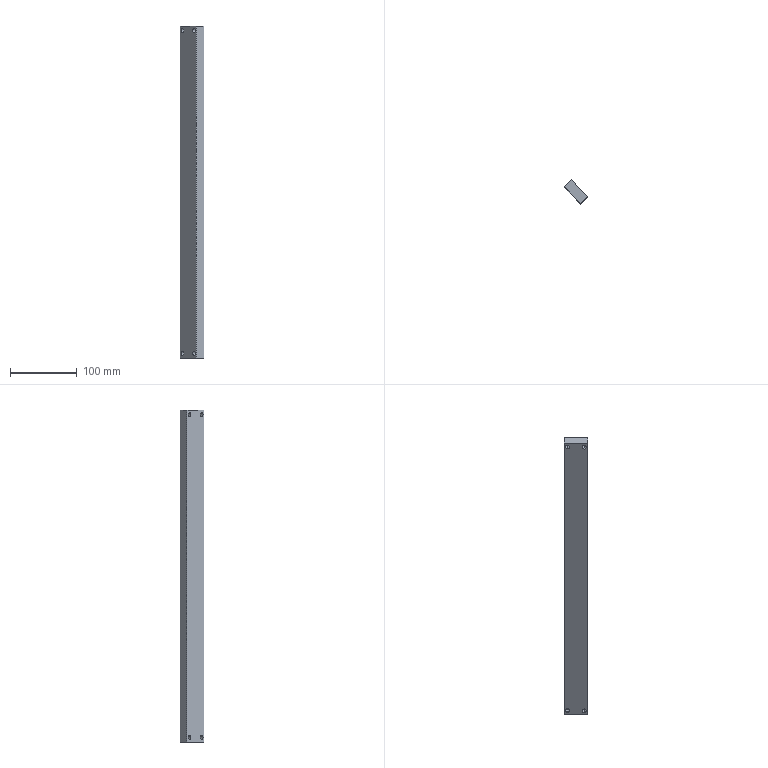Component | SolidWorks | ConnectingPlate-1 | 1 solid | 14 faces | box 34.91 x 35.77 x 499 mm | volume 259984 mm3 | cylinder 8 | plane 6 | commonest cylinder face diameters 6.5 x8
build123d program:
from build123d import *

# Parameters (mm, degrees)
SKETCH1_W           = 499
SKETCH1_H           = 35
SKETCH1_R           = 3.25
BOSS_EXTRUDE1_DEPTH = 15


with BuildPart() as part:
    # Sketch1 → Boss-Extrude1 (new body)
    with BuildSketch(Plane(origin=(0, 0, -7.5), x_dir=(-1, 0, 0), z_dir=(0, 0, -1))):
        Rectangle(SKETCH1_W, SKETCH1_H)
        with Locations(Location((-242.5, 12.5, 0), (0, 0, 180))):
            Circle(SKETCH1_R, mode=Mode.SUBTRACT)
        with Locations(Location((242.5, 12.5, 0), (0, 0, 180))):
            Circle(SKETCH1_R, mode=Mode.SUBTRACT)
        with Locations(Location((242.5, -12.5, 0), (0, 0, 180))):
            Circle(SKETCH1_R, mode=Mode.SUBTRACT)
        with Locations(Location((-242.5, -12.5, 0), (0, 0, 180))):
            Circle(SKETCH1_R, mode=Mode.SUBTRACT)
    extrude(amount=-BOSS_EXTRUDE1_DEPTH)


solid = part.part

# Placed as in the assembly
solid = solid.moved(Location((325.391, 503.025, 0.3), (90, -46.734, 90)))
STEP:
#1=COLOUR_RGB('',0.7922,0.8196,0.9333);
#2=FILL_AREA_STYLE_COLOUR('',#1);
#3=FILL_AREA_STYLE('',(#2));
#4=SURFACE_STYLE_FILL_AREA(#3);
#5=SURFACE_SIDE_STYLE('',(#4));
#6=SURFACE_STYLE_USAGE(.BOTH.,#5);
#7=PRESENTATION_STYLE_ASSIGNMENT((#6));
#8=CARTESIAN_POINT('',(12.933,19.243,9.687));
#9=VERTEX_POINT('',#8);
#10=CARTESIAN_POINT('',(12.933,19.243,9.431));
#11=VERTEX_POINT('',#10);
#12=CARTESIAN_POINT('',(12.933,19.243,9.559));
#13=DIRECTION('',(0.7282,0.6854,-0.));
#14=DIRECTION('',(0.,0.,1.));
#15=AXIS2_PLACEMENT_3D('',#12,#13,#14);
#16=CIRCLE('',#15,0.128);
#17=EDGE_CURVE('',#9,#11,#16,.T.);
#18=ORIENTED_EDGE('',*,*,#17,.F.);
#19=CARTESIAN_POINT('',(13.363,19.648,9.687));
#20=VERTEX_POINT('',#19);
#21=CARTESIAN_POINT('',(12.933,19.243,9.687));
#22=DIRECTION('',(0.7282,0.6854,-0.));
#23=VECTOR('',#22,39.37);
#24=LINE('',#21,#23);
#25=EDGE_CURVE('',#9,#20,#24,.T.);
#26=ORIENTED_EDGE('',*,*,#25,.T.);
#27=CARTESIAN_POINT('',(13.363,19.648,9.431));
#28=VERTEX_POINT('',#27);
#29=CARTESIAN_POINT('',(13.363,19.648,9.559));
#30=DIRECTION('',(0.7282,0.6854,-0.));
#31=DIRECTION('',(0.,0.,1.));
#32=AXIS2_PLACEMENT_3D('',#29,#30,#31);
#33=CIRCLE('',#32,0.128);
#34=EDGE_CURVE('',#20,#28,#33,.T.);
#35=ORIENTED_EDGE('',*,*,#34,.T.);
#36=CARTESIAN_POINT('',(12.933,19.243,9.431));
#37=DIRECTION('',(0.7282,0.6854,-0.));
#38=VECTOR('',#37,39.37);
#39=LINE('',#36,#38);
#40=EDGE_CURVE('',#11,#28,#39,.T.);
#41=ORIENTED_EDGE('',*,*,#40,.F.);
#42=EDGE_LOOP('',(#18,#26,#35,#41));
#43=FACE_OUTER_BOUND('',#42,.T.);
#44=CARTESIAN_POINT('',(12.933,19.243,9.559));
#45=DIRECTION('',(0.7282,0.6854,-0.));
#46=DIRECTION('',(0.,0.,-1.));
#47=AXIS2_PLACEMENT_3D('',#44,#45,#46);
#48=CYLINDRICAL_SURFACE('',#47,0.128);
#49=ADVANCED_FACE('',(#43),#48,.F.);
#50=CARTESIAN_POINT('',(12.933,19.243,-9.407));
#51=VERTEX_POINT('',#50);
#52=CARTESIAN_POINT('',(12.933,19.243,-9.663));
#53=VERTEX_POINT('',#52);
#54=CARTESIAN_POINT('',(12.933,19.243,-9.535));
#55=DIRECTION('',(0.7282,0.6854,-0.));
#56=DIRECTION('',(0.,0.,1.));
#57=AXIS2_PLACEMENT_3D('',#54,#55,#56);
#58=CIRCLE('',#57,0.128);
#59=EDGE_CURVE('',#51,#53,#58,.T.);
#60=ORIENTED_EDGE('',*,*,#59,.F.);
#61=CARTESIAN_POINT('',(13.363,19.648,-9.407));
#62=VERTEX_POINT('',#61);
#63=CARTESIAN_POINT('',(12.933,19.243,-9.407));
#64=DIRECTION('',(0.7282,0.6854,-0.));
#65=VECTOR('',#64,39.37);
#66=LINE('',#63,#65);
#67=EDGE_CURVE('',#51,#62,#66,.T.);
#68=ORIENTED_EDGE('',*,*,#67,.T.);
#69=CARTESIAN_POINT('',(13.363,19.648,-9.663));
#70=VERTEX_POINT('',#69);
#71=CARTESIAN_POINT('',(13.363,19.648,-9.535));
#72=DIRECTION('',(0.7282,0.6854,-0.));
#73=DIRECTION('',(0.,0.,1.));
#74=AXIS2_PLACEMENT_3D('',#71,#72,#73);
#75=CIRCLE('',#74,0.128);
#76=EDGE_CURVE('',#62,#70,#75,.T.);
#77=ORIENTED_EDGE('',*,*,#76,.T.);
#78=CARTESIAN_POINT('',(12.933,19.243,-9.663));
#79=DIRECTION('',(0.7282,0.6854,-0.));
#80=VECTOR('',#79,39.37);
#81=LINE('',#78,#80);
#82=EDGE_CURVE('',#53,#70,#81,.T.);
#83=ORIENTED_EDGE('',*,*,#82,.F.);
#84=EDGE_LOOP('',(#60,#68,#77,#83));
#85=FACE_OUTER_BOUND('',#84,.T.);
#86=CARTESIAN_POINT('',(12.933,19.243,-9.535));
#87=DIRECTION('',(0.7282,0.6854,-0.));
#88=DIRECTION('',(0.,0.,-1.));
#89=AXIS2_PLACEMENT_3D('',#86,#87,#88);
#90=CYLINDRICAL_SURFACE('',#89,0.128);
#91=ADVANCED_FACE('',(#85),#90,.F.);
#92=CARTESIAN_POINT('',(12.258,19.96,-9.407));
#93=VERTEX_POINT('',#92);
#94=CARTESIAN_POINT('',(12.258,19.96,-9.663));
#95=VERTEX_POINT('',#94);
#96=CARTESIAN_POINT('',(12.258,19.96,-9.535));
#97=DIRECTION('',(0.7282,0.6854,-0.));
#98=DIRECTION('',(0.,0.,1.));
#99=AXIS2_PLACEMENT_3D('',#96,#97,#98);
#100=CIRCLE('',#99,0.128);
#101=EDGE_CURVE('',#93,#95,#100,.T.);
#102=ORIENTED_EDGE('',*,*,#101,.F.);
#103=CARTESIAN_POINT('',(12.688,20.365,-9.407));
#104=VERTEX_POINT('',#103);
#105=CARTESIAN_POINT('',(12.258,19.96,-9.407));
#106=DIRECTION('',(0.7282,0.6854,-0.));
#107=VECTOR('',#106,39.37);
#108=LINE('',#105,#107);
#109=EDGE_CURVE('',#93,#104,#108,.T.);
#110=ORIENTED_EDGE('',*,*,#109,.T.);
#111=CARTESIAN_POINT('',(12.688,20.365,-9.663));
#112=VERTEX_POINT('',#111);
#113=CARTESIAN_POINT('',(12.688,20.365,-9.535));
#114=DIRECTION('',(0.7282,0.6854,-0.));
#115=DIRECTION('',(0.,0.,1.));
#116=AXIS2_PLACEMENT_3D('',#113,#114,#115);
#117=CIRCLE('',#116,0.128);
#118=EDGE_CURVE('',#104,#112,#117,.T.);
#119=ORIENTED_EDGE('',*,*,#118,.T.);
#120=CARTESIAN_POINT('',(12.258,19.96,-9.663));
#121=DIRECTION('',(0.7282,0.6854,-0.));
#122=VECTOR('',#121,39.37);
#123=LINE('',#120,#122);
#124=EDGE_CURVE('',#95,#112,#123,.T.);
#125=ORIENTED_EDGE('',*,*,#124,.F.);
#126=EDGE_LOOP('',(#102,#110,#119,#125));
#127=FACE_OUTER_BOUND('',#126,.T.);
#128=CARTESIAN_POINT('',(12.258,19.96,-9.535));
#129=DIRECTION('',(0.7282,0.6854,-0.));
#130=DIRECTION('',(0.,0.,-1.));
#131=AXIS2_PLACEMENT_3D('',#128,#129,#130);
#132=CYLINDRICAL_SURFACE('',#131,0.128);
#133=ADVANCED_FACE('',(#127),#132,.F.);
#134=CARTESIAN_POINT('',(12.258,19.96,9.687));
#135=VERTEX_POINT('',#134);
#136=CARTESIAN_POINT('',(12.258,19.96,9.431));
#137=VERTEX_POINT('',#136);
#138=CARTESIAN_POINT('',(12.258,19.96,9.559));
#139=DIRECTION('',(0.7282,0.6854,-0.));
#140=DIRECTION('',(0.,0.,1.));
#141=AXIS2_PLACEMENT_3D('',#138,#139,#140);
#142=CIRCLE('',#141,0.128);
#143=EDGE_CURVE('',#135,#137,#142,.T.);
#144=ORIENTED_EDGE('',*,*,#143,.F.);
#145=CARTESIAN_POINT('',(12.688,20.365,9.687));
#146=VERTEX_POINT('',#145);
#147=CARTESIAN_POINT('',(12.258,19.96,9.687));
#148=DIRECTION('',(0.7282,0.6854,-0.));
#149=VECTOR('',#148,39.37);
#150=LINE('',#147,#149);
#151=EDGE_CURVE('',#135,#146,#150,.T.);
#152=ORIENTED_EDGE('',*,*,#151,.T.);
#153=CARTESIAN_POINT('',(12.688,20.365,9.431));
#154=VERTEX_POINT('',#153);
#155=CARTESIAN_POINT('',(12.688,20.365,9.559));
#156=DIRECTION('',(0.7282,0.6854,-0.));
#157=DIRECTION('',(0.,0.,1.));
#158=AXIS2_PLACEMENT_3D('',#155,#156,#157);
#159=CIRCLE('',#158,0.128);
#160=EDGE_CURVE('',#146,#154,#159,.T.);
#161=ORIENTED_EDGE('',*,*,#160,.T.);
#162=CARTESIAN_POINT('',(12.258,19.96,9.431));
#163=DIRECTION('',(0.7282,0.6854,-0.));
#164=VECTOR('',#163,39.37);
#165=LINE('',#162,#164);
#166=EDGE_CURVE('',#137,#154,#165,.T.);
#167=ORIENTED_EDGE('',*,*,#166,.F.);
#168=EDGE_LOOP('',(#144,#152,#161,#167));
#169=FACE_OUTER_BOUND('',#168,.T.);
#170=CARTESIAN_POINT('',(12.258,19.96,9.559));
#171=DIRECTION('',(0.7282,0.6854,-0.));
#172=DIRECTION('',(0.,0.,-1.));
#173=AXIS2_PLACEMENT_3D('',#170,#171,#172);
#174=CYLINDRICAL_SURFACE('',#173,0.128);
#175=ADVANCED_FACE('',(#169),#174,.F.);
#176=CARTESIAN_POINT('',(13.498,19.505,9.835));
#177=VERTEX_POINT('',#176);
#178=CARTESIAN_POINT('',(13.498,19.505,-9.811));
#179=VERTEX_POINT('',#178);
#180=CARTESIAN_POINT('',(13.498,19.505,9.835));
#181=DIRECTION('',(0.,-0.,-1.));
#182=VECTOR('',#181,39.37);
#183=LINE('',#180,#182);
#184=EDGE_CURVE('',#177,#179,#183,.T.);
#185=ORIENTED_EDGE('',*,*,#184,.F.);
#186=CARTESIAN_POINT('',(13.068,19.1,9.835));
#187=VERTEX_POINT('',#186);
#188=CARTESIAN_POINT('',(13.068,19.1,9.835));
#189=DIRECTION('',(0.7282,0.6854,-0.));
#190=VECTOR('',#189,39.37);
#191=LINE('',#188,#190);
#192=EDGE_CURVE('',#187,#177,#191,.T.);
#193=ORIENTED_EDGE('',*,*,#192,.F.);
#194=CARTESIAN_POINT('',(13.068,19.1,-9.811));
#195=VERTEX_POINT('',#194);
#196=CARTESIAN_POINT('',(13.068,19.1,9.835));
#197=DIRECTION('',(0.,-0.,-1.));
#198=VECTOR('',#197,39.37);
#199=LINE('',#196,#198);
#200=EDGE_CURVE('',#187,#195,#199,.T.);
#201=ORIENTED_EDGE('',*,*,#200,.T.);
#202=CARTESIAN_POINT('',(13.068,19.1,-9.811));
#203=DIRECTION('',(0.7282,0.6854,-0.));
#204=VECTOR('',#203,39.37);
#205=LINE('',#202,#204);
#206=EDGE_CURVE('',#195,#179,#205,.T.);
#207=ORIENTED_EDGE('',*,*,#206,.T.);
#208=EDGE_LOOP('',(#185,#193,#201,#207));
#209=FACE_OUTER_BOUND('',#208,.T.);
#210=CARTESIAN_POINT('',(13.068,19.1,9.835));
#211=DIRECTION('',(0.6854,-0.7282,0.));
#212=DIRECTION('',(0.7282,0.6854,-0.));
#213=AXIS2_PLACEMENT_3D('',#210,#211,#212);
#214=PLANE('',#213);
#215=ADVANCED_FACE('',(#209),#214,.T.);
#216=CARTESIAN_POINT('',(12.553,20.508,9.835));
#217=VERTEX_POINT('',#216);
#218=CARTESIAN_POINT('',(12.553,20.508,9.835));
#219=DIRECTION('',(0.6854,-0.7282,0.));
#220=VECTOR('',#219,39.37);
#221=LINE('',#218,#220);
#222=EDGE_CURVE('',#217,#177,#221,.T.);
#223=ORIENTED_EDGE('',*,*,#222,.F.);
#224=CARTESIAN_POINT('',(12.123,20.103,9.835));
#225=VERTEX_POINT('',#224);
#226=CARTESIAN_POINT('',(12.123,20.103,9.835));
#227=DIRECTION('',(0.7282,0.6854,-0.));
#228=VECTOR('',#227,39.37);
#229=LINE('',#226,#228);
#230=EDGE_CURVE('',#225,#217,#229,.T.);
#231=ORIENTED_EDGE('',*,*,#230,.F.);
#232=CARTESIAN_POINT('',(12.123,20.103,9.835));
#233=DIRECTION('',(0.6854,-0.7282,0.));
#234=VECTOR('',#233,39.37);
#235=LINE('',#232,#234);
#236=EDGE_CURVE('',#225,#187,#235,.T.);
#237=ORIENTED_EDGE('',*,*,#236,.T.);
#238=ORIENTED_EDGE('',*,*,#192,.T.);
#239=EDGE_LOOP('',(#223,#231,#237,#238));
#240=FACE_OUTER_BOUND('',#239,.T.);
#241=CARTESIAN_POINT('',(12.123,20.103,9.835));
#242=DIRECTION('',(-0.,0.,1.));
#243=DIRECTION('',(0.7282,0.6854,-0.));
#244=AXIS2_PLACEMENT_3D('',#241,#242,#243);
#245=PLANE('',#244);
#246=ADVANCED_FACE('',(#240),#245,.T.);
#247=CARTESIAN_POINT('',(12.553,20.508,-9.811));
#248=VERTEX_POINT('',#247);
#249=CARTESIAN_POINT('',(12.553,20.508,-9.811));
#250=DIRECTION('',(-0.,0.,1.));
#251=VECTOR('',#250,39.37);
#252=LINE('',#249,#251);
#253=EDGE_CURVE('',#248,#217,#252,.T.);
#254=ORIENTED_EDGE('',*,*,#253,.F.);
#255=CARTESIAN_POINT('',(12.123,20.103,-9.811));
#256=VERTEX_POINT('',#255);
#257=CARTESIAN_POINT('',(12.123,20.103,-9.811));
#258=DIRECTION('',(0.7282,0.6854,-0.));
#259=VECTOR('',#258,39.37);
#260=LINE('',#257,#259);
#261=EDGE_CURVE('',#256,#248,#260,.T.);
#262=ORIENTED_EDGE('',*,*,#261,.F.);
#263=CARTESIAN_POINT('',(12.123,20.103,-9.811));
#264=DIRECTION('',(-0.,0.,1.));
#265=VECTOR('',#264,39.37);
#266=LINE('',#263,#265);
#267=EDGE_CURVE('',#256,#225,#266,.T.);
#268=ORIENTED_EDGE('',*,*,#267,.T.);
#269=ORIENTED_EDGE('',*,*,#230,.T.);
#270=EDGE_LOOP('',(#254,#262,#268,#269));
#271=FACE_OUTER_BOUND('',#270,.T.);
#272=CARTESIAN_POINT('',(12.123,20.103,-9.811));
#273=DIRECTION('',(-0.6854,0.7282,-0.));
#274=DIRECTION('',(-0.7282,-0.6854,0.));
#275=AXIS2_PLACEMENT_3D('',#272,#273,#274);
#276=PLANE('',#275);
#277=ADVANCED_FACE('',(#271),#276,.T.);
#278=CARTESIAN_POINT('',(13.498,19.505,-9.811));
#279=DIRECTION('',(-0.6854,0.7282,-0.));
#280=VECTOR('',#279,39.37);
#281=LINE('',#278,#280);
#282=EDGE_CURVE('',#179,#248,#281,.T.);
#283=ORIENTED_EDGE('',*,*,#282,.F.);
#284=ORIENTED_EDGE('',*,*,#206,.F.);
#285=CARTESIAN_POINT('',(13.068,19.1,-9.811));
#286=DIRECTION('',(-0.6854,0.7282,-0.));
#287=VECTOR('',#286,39.37);
#288=LINE('',#285,#287);
#289=EDGE_CURVE('',#195,#256,#288,.T.);
#290=ORIENTED_EDGE('',*,*,#289,.T.);
#291=ORIENTED_EDGE('',*,*,#261,.T.);
#292=EDGE_LOOP('',(#283,#284,#290,#291));
#293=FACE_OUTER_BOUND('',#292,.T.);
#294=CARTESIAN_POINT('',(13.068,19.1,-9.811));
#295=DIRECTION('',(0.,-0.,-1.));
#296=DIRECTION('',(-0.7282,-0.6854,0.));
#297=AXIS2_PLACEMENT_3D('',#294,#295,#296);
#298=PLANE('',#297);
#299=ADVANCED_FACE('',(#293),#298,.T.);
#300=CARTESIAN_POINT('',(12.933,19.243,9.559));
#301=DIRECTION('',(0.7282,0.6854,-0.));
#302=DIRECTION('',(0.,0.,1.));
#303=AXIS2_PLACEMENT_3D('',#300,#301,#302);
#304=CIRCLE('',#303,0.128);
#305=EDGE_CURVE('',#11,#9,#304,.T.);
#306=ORIENTED_EDGE('',*,*,#305,.T.);
#307=ORIENTED_EDGE('',*,*,#17,.T.);
#308=EDGE_LOOP('',(#306,#307));
#309=FACE_BOUND('',#308,.T.);
#310=CARTESIAN_POINT('',(12.933,19.243,-9.535));
#311=DIRECTION('',(0.7282,0.6854,-0.));
#312=DIRECTION('',(0.,0.,1.));
#313=AXIS2_PLACEMENT_3D('',#310,#311,#312);
#314=CIRCLE('',#313,0.128);
#315=EDGE_CURVE('',#53,#51,#314,.T.);
#316=ORIENTED_EDGE('',*,*,#315,.T.);
#317=ORIENTED_EDGE('',*,*,#59,.T.);
#318=EDGE_LOOP('',(#316,#317));
#319=FACE_BOUND('',#318,.T.);
#320=CARTESIAN_POINT('',(12.258,19.96,-9.535));
#321=DIRECTION('',(0.7282,0.6854,-0.));
#322=DIRECTION('',(0.,0.,1.));
#323=AXIS2_PLACEMENT_3D('',#320,#321,#322);
#324=CIRCLE('',#323,0.128);
#325=EDGE_CURVE('',#95,#93,#324,.T.);
#326=ORIENTED_EDGE('',*,*,#325,.T.);
#327=ORIENTED_EDGE('',*,*,#101,.T.);
#328=EDGE_LOOP('',(#326,#327));
#329=FACE_BOUND('',#328,.T.);
#330=CARTESIAN_POINT('',(12.258,19.96,9.559));
#331=DIRECTION('',(0.7282,0.6854,-0.));
#332=DIRECTION('',(0.,0.,1.));
#333=AXIS2_PLACEMENT_3D('',#330,#331,#332);
#334=CIRCLE('',#333,0.128);
#335=EDGE_CURVE('',#137,#135,#334,.T.);
#336=ORIENTED_EDGE('',*,*,#335,.T.);
#337=ORIENTED_EDGE('',*,*,#143,.T.);
#338=EDGE_LOOP('',(#336,#337));
#339=FACE_BOUND('',#338,.T.);
#340=ORIENTED_EDGE('',*,*,#200,.F.);
#341=ORIENTED_EDGE('',*,*,#236,.F.);
#342=ORIENTED_EDGE('',*,*,#267,.F.);
#343=ORIENTED_EDGE('',*,*,#289,.F.);
#344=EDGE_LOOP('',(#340,#341,#342,#343));
#345=FACE_OUTER_BOUND('',#344,.T.);
#346=CARTESIAN_POINT('',(12.596,19.602,0.01181));
#347=DIRECTION('',(0.7282,0.6854,-0.));
#348=DIRECTION('',(0.,-0.,-1.));
#349=AXIS2_PLACEMENT_3D('',#346,#347,#348);
#350=PLANE('',#349);
#351=ADVANCED_FACE('',(#309,#319,#329,#339,#345),#350,.F.);
#352=CARTESIAN_POINT('',(13.363,19.648,9.559));
#353=DIRECTION('',(0.7282,0.6854,-0.));
#354=DIRECTION('',(0.,0.,1.));
#355=AXIS2_PLACEMENT_3D('',#352,#353,#354);
#356=CIRCLE('',#355,0.128);
#357=EDGE_CURVE('',#28,#20,#356,.T.);
#358=ORIENTED_EDGE('',*,*,#357,.F.);
#359=ORIENTED_EDGE('',*,*,#34,.F.);
#360=EDGE_LOOP('',(#358,#359));
#361=FACE_BOUND('',#360,.T.);
#362=CARTESIAN_POINT('',(13.363,19.648,-9.535));
#363=DIRECTION('',(0.7282,0.6854,-0.));
#364=DIRECTION('',(0.,0.,1.));
#365=AXIS2_PLACEMENT_3D('',#362,#363,#364);
#366=CIRCLE('',#365,0.128);
#367=EDGE_CURVE('',#70,#62,#366,.T.);
#368=ORIENTED_EDGE('',*,*,#367,.F.);
#369=ORIENTED_EDGE('',*,*,#76,.F.);
#370=EDGE_LOOP('',(#368,#369));
#371=FACE_BOUND('',#370,.T.);
#372=CARTESIAN_POINT('',(12.688,20.365,-9.535));
#373=DIRECTION('',(0.7282,0.6854,-0.));
#374=DIRECTION('',(0.,0.,1.));
#375=AXIS2_PLACEMENT_3D('',#372,#373,#374);
#376=CIRCLE('',#375,0.128);
#377=EDGE_CURVE('',#112,#104,#376,.T.);
#378=ORIENTED_EDGE('',*,*,#377,.F.);
#379=ORIENTED_EDGE('',*,*,#118,.F.);
#380=EDGE_LOOP('',(#378,#379));
#381=FACE_BOUND('',#380,.T.);
#382=CARTESIAN_POINT('',(12.688,20.365,9.559));
#383=DIRECTION('',(0.7282,0.6854,-0.));
#384=DIRECTION('',(0.,0.,1.));
#385=AXIS2_PLACEMENT_3D('',#382,#383,#384);
#386=CIRCLE('',#385,0.128);
#387=EDGE_CURVE('',#154,#146,#386,.T.);
#388=ORIENTED_EDGE('',*,*,#387,.F.);
#389=ORIENTED_EDGE('',*,*,#160,.F.);
#390=EDGE_LOOP('',(#388,#389));
#391=FACE_BOUND('',#390,.T.);
#392=ORIENTED_EDGE('',*,*,#184,.T.);
#393=ORIENTED_EDGE('',*,*,#282,.T.);
#394=ORIENTED_EDGE('',*,*,#253,.T.);
#395=ORIENTED_EDGE('',*,*,#222,.T.);
#396=EDGE_LOOP('',(#392,#393,#394,#395));
#397=FACE_OUTER_BOUND('',#396,.T.);
#398=CARTESIAN_POINT('',(13.026,20.006,0.01181));
#399=DIRECTION('',(0.7282,0.6854,-0.));
#400=DIRECTION('',(0.,-0.,-1.));
#401=AXIS2_PLACEMENT_3D('',#398,#399,#400);
#402=PLANE('',#401);
#403=ADVANCED_FACE('',(#361,#371,#381,#391,#397),#402,.T.);
#404=ORIENTED_EDGE('',*,*,#151,.F.);
#405=ORIENTED_EDGE('',*,*,#335,.F.);
#406=ORIENTED_EDGE('',*,*,#166,.T.);
#407=ORIENTED_EDGE('',*,*,#387,.T.);
#408=EDGE_LOOP('',(#404,#405,#406,#407));
#409=FACE_OUTER_BOUND('',#408,.T.);
#410=CARTESIAN_POINT('',(12.258,19.96,9.559));
#411=DIRECTION('',(0.7282,0.6854,-0.));
#412=DIRECTION('',(0.,0.,-1.));
#413=AXIS2_PLACEMENT_3D('',#410,#411,#412);
#414=CYLINDRICAL_SURFACE('',#413,0.128);
#415=ADVANCED_FACE('',(#409),#414,.F.);
#416=ORIENTED_EDGE('',*,*,#109,.F.);
#417=ORIENTED_EDGE('',*,*,#325,.F.);
#418=ORIENTED_EDGE('',*,*,#124,.T.);
#419=ORIENTED_EDGE('',*,*,#377,.T.);
#420=EDGE_LOOP('',(#416,#417,#418,#419));
#421=FACE_OUTER_BOUND('',#420,.T.);
#422=CARTESIAN_POINT('',(12.258,19.96,-9.535));
#423=DIRECTION('',(0.7282,0.6854,-0.));
#424=DIRECTION('',(0.,0.,-1.));
#425=AXIS2_PLACEMENT_3D('',#422,#423,#424);
#426=CYLINDRICAL_SURFACE('',#425,0.128);
#427=ADVANCED_FACE('',(#421),#426,.F.);
#428=ORIENTED_EDGE('',*,*,#67,.F.);
#429=ORIENTED_EDGE('',*,*,#315,.F.);
#430=ORIENTED_EDGE('',*,*,#82,.T.);
#431=ORIENTED_EDGE('',*,*,#367,.T.);
#432=EDGE_LOOP('',(#428,#429,#430,#431));
#433=FACE_OUTER_BOUND('',#432,.T.);
#434=CARTESIAN_POINT('',(12.933,19.243,-9.535));
#435=DIRECTION('',(0.7282,0.6854,-0.));
#436=DIRECTION('',(0.,0.,-1.));
#437=AXIS2_PLACEMENT_3D('',#434,#435,#436);
#438=CYLINDRICAL_SURFACE('',#437,0.128);
#439=ADVANCED_FACE('',(#433),#438,.F.);
#440=ORIENTED_EDGE('',*,*,#25,.F.);
#441=ORIENTED_EDGE('',*,*,#305,.F.);
#442=ORIENTED_EDGE('',*,*,#40,.T.);
#443=ORIENTED_EDGE('',*,*,#357,.T.);
#444=EDGE_LOOP('',(#440,#441,#442,#443));
#445=FACE_OUTER_BOUND('',#444,.T.);
#446=CARTESIAN_POINT('',(12.933,19.243,9.559));
#447=DIRECTION('',(0.7282,0.6854,-0.));
#448=DIRECTION('',(0.,0.,-1.));
#449=AXIS2_PLACEMENT_3D('',#446,#447,#448);
#450=CYLINDRICAL_SURFACE('',#449,0.128);
#451=ADVANCED_FACE('',(#445),#450,.F.);
#452=CLOSED_SHELL('',(#49,#91,#133,#175,#215,#246,#277,#299,#351,#403,#415,#427,#439,#451));
#453=MANIFOLD_SOLID_BREP('',#452);
#454=STYLED_ITEM('',(#7),#453);
#455=(LENGTH_UNIT()NAMED_UNIT(*)SI_UNIT($,.METRE.));
#456=LENGTH_MEASURE_WITH_UNIT(LENGTH_MEASURE(0.0254),#455);
#457=DIMENSIONAL_EXPONENTS(1.,0.,0.,0.,0.,0.,0.);
#458=(CONVERSION_BASED_UNIT('',#456)LENGTH_UNIT()NAMED_UNIT(#457));
#459=UNCERTAINTY_MEASURE_WITH_UNIT(LENGTH_MEASURE(0.00001),#458,'','');
#460=(NAMED_UNIT(*)PLANE_ANGLE_UNIT()SI_UNIT($,.RADIAN.));
#461=(NAMED_UNIT(*)SI_UNIT($,.STERADIAN.)SOLID_ANGLE_UNIT());
#462=(GEOMETRIC_REPRESENTATION_CONTEXT(3)GLOBAL_UNCERTAINTY_ASSIGNED_CONTEXT((#459))GLOBAL_UNIT_ASSIGNED_CONTEXT((#458,#460,#461))REPRESENTATION_CONTEXT('',''));
#463=MECHANICAL_DESIGN_GEOMETRIC_PRESENTATION_REPRESENTATION('',(#454),#462);
#464=CARTESIAN_POINT('',(0.,0.,0.));
#465=DIRECTION('',(0.,0.,1.));
#466=DIRECTION('',(1.,0.,0.));
#467=AXIS2_PLACEMENT_3D('',#464,#465,#466);
#468=(LENGTH_UNIT()NAMED_UNIT(*)SI_UNIT($,.METRE.));
#469=LENGTH_MEASURE_WITH_UNIT(LENGTH_MEASURE(0.0254),#468);
#470=DIMENSIONAL_EXPONENTS(1.,0.,0.,0.,0.,0.,0.);
#471=(CONVERSION_BASED_UNIT('',#469)LENGTH_UNIT()NAMED_UNIT(#470));
#472=UNCERTAINTY_MEASURE_WITH_UNIT(LENGTH_MEASURE(0.00001),#471,'','');
#473=(NAMED_UNIT(*)PLANE_ANGLE_UNIT()SI_UNIT($,.RADIAN.));
#474=(NAMED_UNIT(*)SI_UNIT($,.STERADIAN.)SOLID_ANGLE_UNIT());
#475=(GEOMETRIC_REPRESENTATION_CONTEXT(3)GLOBAL_UNCERTAINTY_ASSIGNED_CONTEXT((#472))GLOBAL_UNIT_ASSIGNED_CONTEXT((#471,#473,#474))REPRESENTATION_CONTEXT('',''));
#476=ADVANCED_BREP_SHAPE_REPRESENTATION('',(#453,#467),#475);
#477=PRESENTATION_LAYER_ASSIGNMENT('','',(#454));